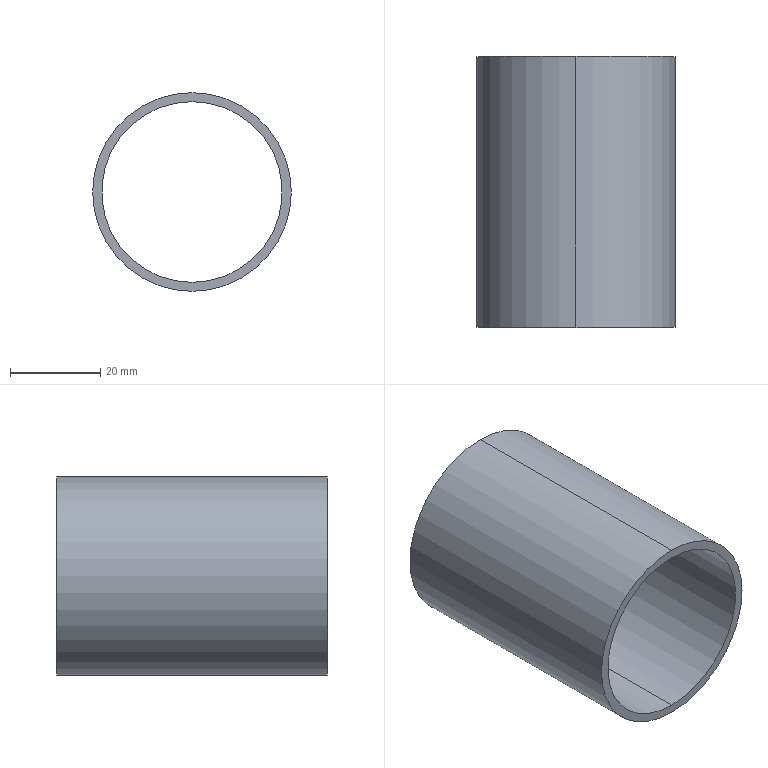Component | SolidWorks | GuideSleeve-1 | 1 solid | 6 faces | box 44 x 60 x 44 mm | volume 15834 mm3 | cylinder 4 | plane 2 | commonest cylinder face diameters 40 x2 44 x2
build123d program:
from build123d import *

# Parameters (mm, degrees)
SKETCH1_R           = 22
SKETCH1_R_2         = 20
BOSS_EXTRUDE1_DEPTH = 60


with BuildPart() as part:
    # Sketch1 → Boss-Extrude1 (new body)
    with BuildSketch(Plane(origin=(0, 0, 0), x_dir=(1, 0, 0), z_dir=(0, 1, 0))):
        with Locations(Location((0, 0, 0), (0, 0, 270))):
            Circle(SKETCH1_R)
        with Locations(Location((0, 0, 0), (0, 0, 270))):
            Circle(SKETCH1_R_2, mode=Mode.SUBTRACT)
    extrude(amount=BOSS_EXTRUDE1_DEPTH)


solid = part.part

# Placed as in the assembly
solid = solid.moved(Location((135.493, -66.411, 458), (0, 0, 0)))
STEP:
#1=COLOUR_RGB('',0.7922,0.8196,0.9333);
#2=FILL_AREA_STYLE_COLOUR('',#1);
#3=FILL_AREA_STYLE('',(#2));
#4=SURFACE_STYLE_FILL_AREA(#3);
#5=SURFACE_SIDE_STYLE('',(#4));
#6=SURFACE_STYLE_USAGE(.BOTH.,#5);
#7=PRESENTATION_STYLE_ASSIGNMENT((#6));
#8=CARTESIAN_POINT('',(5.334,-0.2524,17.244));
#9=VERTEX_POINT('',#8);
#10=CARTESIAN_POINT('',(5.334,-0.2524,18.819));
#11=VERTEX_POINT('',#10);
#12=CARTESIAN_POINT('',(5.334,-0.2524,18.031));
#13=DIRECTION('',(0.,1.,0.));
#14=DIRECTION('',(0.,0.,1.));
#15=AXIS2_PLACEMENT_3D('',#12,#13,#14);
#16=CIRCLE('',#15,0.7874);
#17=EDGE_CURVE('',#9,#11,#16,.T.);
#18=ORIENTED_EDGE('',*,*,#17,.T.);
#19=CARTESIAN_POINT('',(5.334,-2.615,18.819));
#20=VERTEX_POINT('',#19);
#21=CARTESIAN_POINT('',(5.334,-0.2524,18.819));
#22=DIRECTION('',(0.,-1.,0.));
#23=VECTOR('',#22,39.37);
#24=LINE('',#21,#23);
#25=EDGE_CURVE('',#11,#20,#24,.T.);
#26=ORIENTED_EDGE('',*,*,#25,.T.);
#27=CARTESIAN_POINT('',(5.334,-2.615,17.244));
#28=VERTEX_POINT('',#27);
#29=CARTESIAN_POINT('',(5.334,-2.615,18.031));
#30=DIRECTION('',(0.,1.,0.));
#31=DIRECTION('',(0.,0.,1.));
#32=AXIS2_PLACEMENT_3D('',#29,#30,#31);
#33=CIRCLE('',#32,0.7874);
#34=EDGE_CURVE('',#28,#20,#33,.T.);
#35=ORIENTED_EDGE('',*,*,#34,.F.);
#36=CARTESIAN_POINT('',(5.334,-0.2524,17.244));
#37=DIRECTION('',(0.,-1.,0.));
#38=VECTOR('',#37,39.37);
#39=LINE('',#36,#38);
#40=EDGE_CURVE('',#9,#28,#39,.T.);
#41=ORIENTED_EDGE('',*,*,#40,.F.);
#42=EDGE_LOOP('',(#18,#26,#35,#41));
#43=FACE_OUTER_BOUND('',#42,.T.);
#44=CARTESIAN_POINT('',(5.334,-0.2524,18.031));
#45=DIRECTION('',(0.,-1.,0.));
#46=DIRECTION('',(0.,0.,-1.));
#47=AXIS2_PLACEMENT_3D('',#44,#45,#46);
#48=CYLINDRICAL_SURFACE('',#47,0.7874);
#49=ADVANCED_FACE('',(#43),#48,.F.);
#50=CARTESIAN_POINT('',(5.334,-0.2524,18.898));
#51=VERTEX_POINT('',#50);
#52=CARTESIAN_POINT('',(5.334,-0.2524,17.165));
#53=VERTEX_POINT('',#52);
#54=CARTESIAN_POINT('',(5.334,-0.2524,18.031));
#55=DIRECTION('',(0.,1.,0.));
#56=DIRECTION('',(0.,0.,1.));
#57=AXIS2_PLACEMENT_3D('',#54,#55,#56);
#58=CIRCLE('',#57,0.8661);
#59=EDGE_CURVE('',#51,#53,#58,.T.);
#60=ORIENTED_EDGE('',*,*,#59,.F.);
#61=CARTESIAN_POINT('',(5.334,-2.615,18.898));
#62=VERTEX_POINT('',#61);
#63=CARTESIAN_POINT('',(5.334,-0.2524,18.898));
#64=DIRECTION('',(0.,-1.,0.));
#65=VECTOR('',#64,39.37);
#66=LINE('',#63,#65);
#67=EDGE_CURVE('',#51,#62,#66,.T.);
#68=ORIENTED_EDGE('',*,*,#67,.T.);
#69=CARTESIAN_POINT('',(5.334,-2.615,17.165));
#70=VERTEX_POINT('',#69);
#71=CARTESIAN_POINT('',(5.334,-2.615,18.031));
#72=DIRECTION('',(0.,1.,0.));
#73=DIRECTION('',(0.,0.,1.));
#74=AXIS2_PLACEMENT_3D('',#71,#72,#73);
#75=CIRCLE('',#74,0.8661);
#76=EDGE_CURVE('',#62,#70,#75,.T.);
#77=ORIENTED_EDGE('',*,*,#76,.T.);
#78=CARTESIAN_POINT('',(5.334,-0.2524,17.165));
#79=DIRECTION('',(0.,-1.,0.));
#80=VECTOR('',#79,39.37);
#81=LINE('',#78,#80);
#82=EDGE_CURVE('',#53,#70,#81,.T.);
#83=ORIENTED_EDGE('',*,*,#82,.F.);
#84=EDGE_LOOP('',(#60,#68,#77,#83));
#85=FACE_OUTER_BOUND('',#84,.T.);
#86=CARTESIAN_POINT('',(5.334,-0.2524,18.031));
#87=DIRECTION('',(0.,-1.,0.));
#88=DIRECTION('',(0.,0.,-1.));
#89=AXIS2_PLACEMENT_3D('',#86,#87,#88);
#90=CYLINDRICAL_SURFACE('',#89,0.8661);
#91=ADVANCED_FACE('',(#85),#90,.T.);
#92=CARTESIAN_POINT('',(5.334,-0.2524,18.031));
#93=DIRECTION('',(0.,1.,0.));
#94=DIRECTION('',(0.,0.,1.));
#95=AXIS2_PLACEMENT_3D('',#92,#93,#94);
#96=CIRCLE('',#95,0.8661);
#97=EDGE_CURVE('',#53,#51,#96,.T.);
#98=ORIENTED_EDGE('',*,*,#97,.T.);
#99=ORIENTED_EDGE('',*,*,#59,.T.);
#100=EDGE_LOOP('',(#98,#99));
#101=FACE_OUTER_BOUND('',#100,.T.);
#102=ORIENTED_EDGE('',*,*,#17,.F.);
#103=CARTESIAN_POINT('',(5.334,-0.2524,18.031));
#104=DIRECTION('',(0.,1.,0.));
#105=DIRECTION('',(0.,0.,1.));
#106=AXIS2_PLACEMENT_3D('',#103,#104,#105);
#107=CIRCLE('',#106,0.7874);
#108=EDGE_CURVE('',#11,#9,#107,.T.);
#109=ORIENTED_EDGE('',*,*,#108,.F.);
#110=EDGE_LOOP('',(#102,#109));
#111=FACE_BOUND('',#110,.T.);
#112=CARTESIAN_POINT('',(5.334,-0.2524,18.031));
#113=DIRECTION('',(0.,1.,0.));
#114=DIRECTION('',(0.,0.,1.));
#115=AXIS2_PLACEMENT_3D('',#112,#113,#114);
#116=PLANE('',#115);
#117=ADVANCED_FACE('',(#101,#111),#116,.T.);
#118=CARTESIAN_POINT('',(5.334,-2.615,18.031));
#119=DIRECTION('',(0.,1.,0.));
#120=DIRECTION('',(0.,0.,1.));
#121=AXIS2_PLACEMENT_3D('',#118,#119,#120);
#122=CIRCLE('',#121,0.8661);
#123=EDGE_CURVE('',#70,#62,#122,.T.);
#124=ORIENTED_EDGE('',*,*,#123,.F.);
#125=ORIENTED_EDGE('',*,*,#76,.F.);
#126=EDGE_LOOP('',(#124,#125));
#127=FACE_OUTER_BOUND('',#126,.T.);
#128=ORIENTED_EDGE('',*,*,#34,.T.);
#129=CARTESIAN_POINT('',(5.334,-2.615,18.031));
#130=DIRECTION('',(0.,1.,0.));
#131=DIRECTION('',(0.,0.,1.));
#132=AXIS2_PLACEMENT_3D('',#129,#130,#131);
#133=CIRCLE('',#132,0.7874);
#134=EDGE_CURVE('',#20,#28,#133,.T.);
#135=ORIENTED_EDGE('',*,*,#134,.T.);
#136=EDGE_LOOP('',(#128,#135));
#137=FACE_BOUND('',#136,.T.);
#138=CARTESIAN_POINT('',(5.334,-2.615,18.031));
#139=DIRECTION('',(0.,1.,0.));
#140=DIRECTION('',(0.,0.,1.));
#141=AXIS2_PLACEMENT_3D('',#138,#139,#140);
#142=PLANE('',#141);
#143=ADVANCED_FACE('',(#127,#137),#142,.F.);
#144=ORIENTED_EDGE('',*,*,#67,.F.);
#145=ORIENTED_EDGE('',*,*,#97,.F.);
#146=ORIENTED_EDGE('',*,*,#82,.T.);
#147=ORIENTED_EDGE('',*,*,#123,.T.);
#148=EDGE_LOOP('',(#144,#145,#146,#147));
#149=FACE_OUTER_BOUND('',#148,.T.);
#150=CARTESIAN_POINT('',(5.334,-0.2524,18.031));
#151=DIRECTION('',(0.,-1.,0.));
#152=DIRECTION('',(0.,0.,-1.));
#153=AXIS2_PLACEMENT_3D('',#150,#151,#152);
#154=CYLINDRICAL_SURFACE('',#153,0.8661);
#155=ADVANCED_FACE('',(#149),#154,.T.);
#156=ORIENTED_EDGE('',*,*,#25,.F.);
#157=ORIENTED_EDGE('',*,*,#108,.T.);
#158=ORIENTED_EDGE('',*,*,#40,.T.);
#159=ORIENTED_EDGE('',*,*,#134,.F.);
#160=EDGE_LOOP('',(#156,#157,#158,#159));
#161=FACE_OUTER_BOUND('',#160,.T.);
#162=CARTESIAN_POINT('',(5.334,-0.2524,18.031));
#163=DIRECTION('',(0.,-1.,0.));
#164=DIRECTION('',(0.,0.,-1.));
#165=AXIS2_PLACEMENT_3D('',#162,#163,#164);
#166=CYLINDRICAL_SURFACE('',#165,0.7874);
#167=ADVANCED_FACE('',(#161),#166,.F.);
#168=CLOSED_SHELL('',(#49,#91,#117,#143,#155,#167));
#169=MANIFOLD_SOLID_BREP('',#168);
#170=STYLED_ITEM('',(#7),#169);
#171=PRESENTATION_LAYER_ASSIGNMENT('','',(#170));
#172=CARTESIAN_POINT('',(0.,0.,0.));
#173=DIRECTION('',(0.,0.,1.));
#174=DIRECTION('',(1.,0.,0.));
#175=AXIS2_PLACEMENT_3D('',#172,#173,#174);
#176=(LENGTH_UNIT()NAMED_UNIT(*)SI_UNIT($,.METRE.));
#177=LENGTH_MEASURE_WITH_UNIT(LENGTH_MEASURE(0.0254),#176);
#178=DIMENSIONAL_EXPONENTS(1.,0.,0.,0.,0.,0.,0.);
#179=(CONVERSION_BASED_UNIT('',#177)LENGTH_UNIT()NAMED_UNIT(#178));
#180=UNCERTAINTY_MEASURE_WITH_UNIT(LENGTH_MEASURE(0.00001),#179,'','');
#181=(NAMED_UNIT(*)PLANE_ANGLE_UNIT()SI_UNIT($,.RADIAN.));
#182=(NAMED_UNIT(*)SI_UNIT($,.STERADIAN.)SOLID_ANGLE_UNIT());
#183=(GEOMETRIC_REPRESENTATION_CONTEXT(3)GLOBAL_UNCERTAINTY_ASSIGNED_CONTEXT((#180))GLOBAL_UNIT_ASSIGNED_CONTEXT((#179,#181,#182))REPRESENTATION_CONTEXT('',''));
#184=ADVANCED_BREP_SHAPE_REPRESENTATION('',(#169,#175),#183);
#185=(LENGTH_UNIT()NAMED_UNIT(*)SI_UNIT($,.METRE.));
#186=LENGTH_MEASURE_WITH_UNIT(LENGTH_MEASURE(0.0254),#185);
#187=DIMENSIONAL_EXPONENTS(1.,0.,0.,0.,0.,0.,0.);
#188=(CONVERSION_BASED_UNIT('',#186)LENGTH_UNIT()NAMED_UNIT(#187));
#189=UNCERTAINTY_MEASURE_WITH_UNIT(LENGTH_MEASURE(0.00001),#188,'','');
#190=(NAMED_UNIT(*)PLANE_ANGLE_UNIT()SI_UNIT($,.RADIAN.));
#191=(NAMED_UNIT(*)SI_UNIT($,.STERADIAN.)SOLID_ANGLE_UNIT());
#192=(GEOMETRIC_REPRESENTATION_CONTEXT(3)GLOBAL_UNCERTAINTY_ASSIGNED_CONTEXT((#189))GLOBAL_UNIT_ASSIGNED_CONTEXT((#188,#190,#191))REPRESENTATION_CONTEXT('',''));
#193=MECHANICAL_DESIGN_GEOMETRIC_PRESENTATION_REPRESENTATION('',(#170),#192);